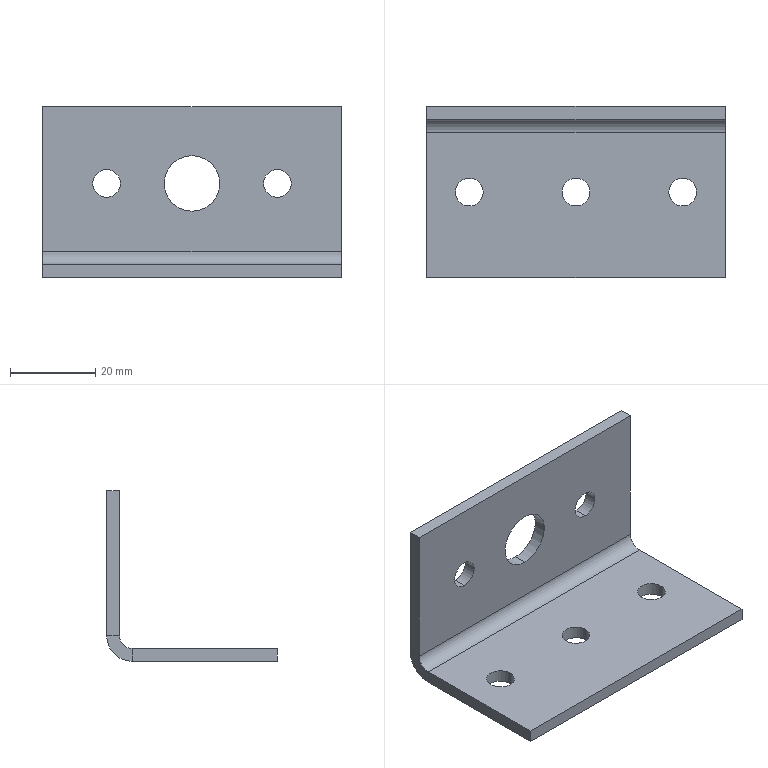Component | SolidWorks | SidePanelAssembly-1_LiftingRingReinforcementPlate-1 | 1 solid | 26 faces | box 70 x 40 x 40 mm | volume 14868 mm3 | cylinder 14 | plane 12 | commonest cylinder face diameters 6.5 x10 13 x2 12 x1 6 x1
STEP:
#1=CARTESIAN_POINT('',(27.472,71.421,-22.766));
#2=VERTEX_POINT('',#1);
#3=CARTESIAN_POINT('',(27.472,71.421,-22.51));
#4=VERTEX_POINT('',#3);
#5=CARTESIAN_POINT('',(27.472,71.421,-22.638));
#6=DIRECTION('',(0.,1.,0.));
#7=DIRECTION('',(0.,0.,1.));
#8=AXIS2_PLACEMENT_3D('',#5,#6,#7);
#9=CIRCLE('',#8,0.128);
#10=EDGE_CURVE('',#2,#4,#9,.T.);
#11=ORIENTED_EDGE('',*,*,#10,.T.);
#12=CARTESIAN_POINT('',(27.472,71.303,-22.51));
#13=VERTEX_POINT('',#12);
#14=CARTESIAN_POINT('',(27.472,71.697,-22.51));
#15=DIRECTION('',(0.,-1.,0.));
#16=VECTOR('',#15,39.37);
#17=LINE('',#14,#16);
#18=EDGE_CURVE('',#4,#13,#17,.T.);
#19=ORIENTED_EDGE('',*,*,#18,.T.);
#20=CARTESIAN_POINT('',(27.472,71.303,-22.766));
#21=VERTEX_POINT('',#20);
#22=CARTESIAN_POINT('',(27.472,71.303,-22.638));
#23=DIRECTION('',(0.,-1.,0.));
#24=DIRECTION('',(0.,0.,-1.));
#25=AXIS2_PLACEMENT_3D('',#22,#23,#24);
#26=CIRCLE('',#25,0.128);
#27=EDGE_CURVE('',#13,#21,#26,.T.);
#28=ORIENTED_EDGE('',*,*,#27,.T.);
#29=CARTESIAN_POINT('',(27.472,71.697,-22.766));
#30=DIRECTION('',(0.,-1.,0.));
#31=VECTOR('',#30,39.37);
#32=LINE('',#29,#31);
#33=EDGE_CURVE('',#2,#21,#32,.T.);
#34=ORIENTED_EDGE('',*,*,#33,.F.);
#35=EDGE_LOOP('',(#11,#19,#28,#34));
#36=FACE_OUTER_BOUND('',#35,.T.);
#37=CARTESIAN_POINT('',(27.472,71.697,-22.638));
#38=DIRECTION('',(0.,-1.,0.));
#39=DIRECTION('',(0.,0.,-1.));
#40=AXIS2_PLACEMENT_3D('',#37,#38,#39);
#41=CYLINDRICAL_SURFACE('',#40,0.128);
#42=ADVANCED_FACE('',(#36),#41,.F.);
#43=CARTESIAN_POINT('',(25.897,71.421,-22.766));
#44=VERTEX_POINT('',#43);
#45=CARTESIAN_POINT('',(25.897,71.421,-22.51));
#46=VERTEX_POINT('',#45);
#47=CARTESIAN_POINT('',(25.897,71.421,-22.638));
#48=DIRECTION('',(0.,1.,0.));
#49=DIRECTION('',(0.,0.,1.));
#50=AXIS2_PLACEMENT_3D('',#47,#48,#49);
#51=CIRCLE('',#50,0.128);
#52=EDGE_CURVE('',#44,#46,#51,.T.);
#53=ORIENTED_EDGE('',*,*,#52,.T.);
#54=CARTESIAN_POINT('',(25.897,71.303,-22.51));
#55=VERTEX_POINT('',#54);
#56=CARTESIAN_POINT('',(25.897,71.697,-22.51));
#57=DIRECTION('',(0.,-1.,0.));
#58=VECTOR('',#57,39.37);
#59=LINE('',#56,#58);
#60=EDGE_CURVE('',#46,#55,#59,.T.);
#61=ORIENTED_EDGE('',*,*,#60,.T.);
#62=CARTESIAN_POINT('',(25.897,71.303,-22.766));
#63=VERTEX_POINT('',#62);
#64=CARTESIAN_POINT('',(25.897,71.303,-22.638));
#65=DIRECTION('',(0.,-1.,0.));
#66=DIRECTION('',(0.,0.,-1.));
#67=AXIS2_PLACEMENT_3D('',#64,#65,#66);
#68=CIRCLE('',#67,0.128);
#69=EDGE_CURVE('',#55,#63,#68,.T.);
#70=ORIENTED_EDGE('',*,*,#69,.T.);
#71=CARTESIAN_POINT('',(25.897,71.697,-22.766));
#72=DIRECTION('',(0.,-1.,0.));
#73=VECTOR('',#72,39.37);
#74=LINE('',#71,#73);
#75=EDGE_CURVE('',#44,#63,#74,.T.);
#76=ORIENTED_EDGE('',*,*,#75,.F.);
#77=EDGE_LOOP('',(#53,#61,#70,#76));
#78=FACE_OUTER_BOUND('',#77,.T.);
#79=CARTESIAN_POINT('',(25.897,71.697,-22.638));
#80=DIRECTION('',(0.,-1.,0.));
#81=DIRECTION('',(0.,0.,-1.));
#82=AXIS2_PLACEMENT_3D('',#79,#80,#81);
#83=CYLINDRICAL_SURFACE('',#82,0.128);
#84=ADVANCED_FACE('',(#78),#83,.F.);
#85=CARTESIAN_POINT('',(27.541,70.634,-23.504));
#86=VERTEX_POINT('',#85);
#87=CARTESIAN_POINT('',(27.797,70.634,-23.504));
#88=VERTEX_POINT('',#87);
#89=CARTESIAN_POINT('',(27.669,70.634,-23.504));
#90=DIRECTION('',(0.,-0.,1.));
#91=DIRECTION('',(0.,-1.,0.));
#92=AXIS2_PLACEMENT_3D('',#89,#90,#91);
#93=CIRCLE('',#92,0.128);
#94=EDGE_CURVE('',#86,#88,#93,.T.);
#95=ORIENTED_EDGE('',*,*,#94,.F.);
#96=CARTESIAN_POINT('',(27.541,70.634,-23.386));
#97=VERTEX_POINT('',#96);
#98=CARTESIAN_POINT('',(27.541,70.634,-23.78));
#99=DIRECTION('',(0.,0.,1.));
#100=VECTOR('',#99,39.37);
#101=LINE('',#98,#100);
#102=EDGE_CURVE('',#86,#97,#101,.T.);
#103=ORIENTED_EDGE('',*,*,#102,.T.);
#104=CARTESIAN_POINT('',(27.797,70.634,-23.386));
#105=VERTEX_POINT('',#104);
#106=CARTESIAN_POINT('',(27.669,70.634,-23.386));
#107=DIRECTION('',(0.,0.,1.));
#108=DIRECTION('',(1.,0.,0.));
#109=AXIS2_PLACEMENT_3D('',#106,#107,#108);
#110=CIRCLE('',#109,0.128);
#111=EDGE_CURVE('',#97,#105,#110,.T.);
#112=ORIENTED_EDGE('',*,*,#111,.T.);
#113=CARTESIAN_POINT('',(27.797,70.634,-23.78));
#114=DIRECTION('',(0.,0.,1.));
#115=VECTOR('',#114,39.37);
#116=LINE('',#113,#115);
#117=EDGE_CURVE('',#88,#105,#116,.T.);
#118=ORIENTED_EDGE('',*,*,#117,.F.);
#119=EDGE_LOOP('',(#95,#103,#112,#118));
#120=FACE_OUTER_BOUND('',#119,.T.);
#121=CARTESIAN_POINT('',(27.669,70.634,-23.78));
#122=DIRECTION('',(0.,0.,1.));
#123=DIRECTION('',(1.,0.,0.));
#124=AXIS2_PLACEMENT_3D('',#121,#122,#123);
#125=CYLINDRICAL_SURFACE('',#124,0.128);
#126=ADVANCED_FACE('',(#120),#125,.F.);
#127=CARTESIAN_POINT('',(26.556,70.634,-23.504));
#128=VERTEX_POINT('',#127);
#129=CARTESIAN_POINT('',(26.812,70.634,-23.504));
#130=VERTEX_POINT('',#129);
#131=CARTESIAN_POINT('',(26.684,70.634,-23.504));
#132=DIRECTION('',(0.,-0.,1.));
#133=DIRECTION('',(0.,-1.,0.));
#134=AXIS2_PLACEMENT_3D('',#131,#132,#133);
#135=CIRCLE('',#134,0.128);
#136=EDGE_CURVE('',#128,#130,#135,.T.);
#137=ORIENTED_EDGE('',*,*,#136,.F.);
#138=CARTESIAN_POINT('',(26.556,70.634,-23.386));
#139=VERTEX_POINT('',#138);
#140=CARTESIAN_POINT('',(26.556,70.634,-23.78));
#141=DIRECTION('',(0.,0.,1.));
#142=VECTOR('',#141,39.37);
#143=LINE('',#140,#142);
#144=EDGE_CURVE('',#128,#139,#143,.T.);
#145=ORIENTED_EDGE('',*,*,#144,.T.);
#146=CARTESIAN_POINT('',(26.812,70.634,-23.386));
#147=VERTEX_POINT('',#146);
#148=CARTESIAN_POINT('',(26.684,70.634,-23.386));
#149=DIRECTION('',(0.,0.,1.));
#150=DIRECTION('',(1.,0.,0.));
#151=AXIS2_PLACEMENT_3D('',#148,#149,#150);
#152=CIRCLE('',#151,0.128);
#153=EDGE_CURVE('',#139,#147,#152,.T.);
#154=ORIENTED_EDGE('',*,*,#153,.T.);
#155=CARTESIAN_POINT('',(26.812,70.634,-23.78));
#156=DIRECTION('',(0.,0.,1.));
#157=VECTOR('',#156,39.37);
#158=LINE('',#155,#157);
#159=EDGE_CURVE('',#130,#147,#158,.T.);
#160=ORIENTED_EDGE('',*,*,#159,.F.);
#161=EDGE_LOOP('',(#137,#145,#154,#160));
#162=FACE_OUTER_BOUND('',#161,.T.);
#163=CARTESIAN_POINT('',(26.684,70.634,-23.78));
#164=DIRECTION('',(0.,0.,1.));
#165=DIRECTION('',(1.,0.,0.));
#166=AXIS2_PLACEMENT_3D('',#163,#164,#165);
#167=CYLINDRICAL_SURFACE('',#166,0.128);
#168=ADVANCED_FACE('',(#162),#167,.F.);
#169=CARTESIAN_POINT('',(25.572,70.634,-23.504));
#170=VERTEX_POINT('',#169);
#171=CARTESIAN_POINT('',(25.828,70.634,-23.504));
#172=VERTEX_POINT('',#171);
#173=CARTESIAN_POINT('',(25.7,70.634,-23.504));
#174=DIRECTION('',(0.,-0.,1.));
#175=DIRECTION('',(0.,-1.,0.));
#176=AXIS2_PLACEMENT_3D('',#173,#174,#175);
#177=CIRCLE('',#176,0.128);
#178=EDGE_CURVE('',#170,#172,#177,.T.);
#179=ORIENTED_EDGE('',*,*,#178,.F.);
#180=CARTESIAN_POINT('',(25.572,70.634,-23.386));
#181=VERTEX_POINT('',#180);
#182=CARTESIAN_POINT('',(25.572,70.634,-23.78));
#183=DIRECTION('',(0.,0.,1.));
#184=VECTOR('',#183,39.37);
#185=LINE('',#182,#184);
#186=EDGE_CURVE('',#170,#181,#185,.T.);
#187=ORIENTED_EDGE('',*,*,#186,.T.);
#188=CARTESIAN_POINT('',(25.828,70.634,-23.386));
#189=VERTEX_POINT('',#188);
#190=CARTESIAN_POINT('',(25.7,70.634,-23.386));
#191=DIRECTION('',(0.,0.,1.));
#192=DIRECTION('',(1.,0.,0.));
#193=AXIS2_PLACEMENT_3D('',#190,#191,#192);
#194=CIRCLE('',#193,0.128);
#195=EDGE_CURVE('',#181,#189,#194,.T.);
#196=ORIENTED_EDGE('',*,*,#195,.T.);
#197=CARTESIAN_POINT('',(25.828,70.634,-23.78));
#198=DIRECTION('',(0.,0.,1.));
#199=VECTOR('',#198,39.37);
#200=LINE('',#197,#199);
#201=EDGE_CURVE('',#172,#189,#200,.T.);
#202=ORIENTED_EDGE('',*,*,#201,.F.);
#203=EDGE_LOOP('',(#179,#187,#196,#202));
#204=FACE_OUTER_BOUND('',#203,.T.);
#205=CARTESIAN_POINT('',(25.7,70.634,-23.78));
#206=DIRECTION('',(0.,0.,1.));
#207=DIRECTION('',(1.,0.,0.));
#208=AXIS2_PLACEMENT_3D('',#205,#206,#207);
#209=CYLINDRICAL_SURFACE('',#208,0.128);
#210=ADVANCED_FACE('',(#204),#209,.F.);
#211=CARTESIAN_POINT('',(26.684,71.303,-22.894));
#212=VERTEX_POINT('',#211);
#213=CARTESIAN_POINT('',(26.684,71.303,-22.382));
#214=VERTEX_POINT('',#213);
#215=CARTESIAN_POINT('',(26.684,71.303,-22.638));
#216=DIRECTION('',(0.,1.,0.));
#217=DIRECTION('',(0.,0.,1.));
#218=AXIS2_PLACEMENT_3D('',#215,#216,#217);
#219=CIRCLE('',#218,0.2559);
#220=EDGE_CURVE('',#212,#214,#219,.T.);
#221=ORIENTED_EDGE('',*,*,#220,.F.);
#222=CARTESIAN_POINT('',(26.684,71.421,-22.894));
#223=VERTEX_POINT('',#222);
#224=CARTESIAN_POINT('',(26.684,71.028,-22.894));
#225=DIRECTION('',(0.,1.,0.));
#226=VECTOR('',#225,39.37);
#227=LINE('',#224,#226);
#228=EDGE_CURVE('',#212,#223,#227,.T.);
#229=ORIENTED_EDGE('',*,*,#228,.T.);
#230=CARTESIAN_POINT('',(26.684,71.421,-22.382));
#231=VERTEX_POINT('',#230);
#232=CARTESIAN_POINT('',(26.684,71.421,-22.638));
#233=DIRECTION('',(0.,1.,0.));
#234=DIRECTION('',(0.,0.,1.));
#235=AXIS2_PLACEMENT_3D('',#232,#233,#234);
#236=CIRCLE('',#235,0.2559);
#237=EDGE_CURVE('',#223,#231,#236,.T.);
#238=ORIENTED_EDGE('',*,*,#237,.T.);
#239=CARTESIAN_POINT('',(26.684,71.028,-22.382));
#240=DIRECTION('',(0.,1.,0.));
#241=VECTOR('',#240,39.37);
#242=LINE('',#239,#241);
#243=EDGE_CURVE('',#214,#231,#242,.T.);
#244=ORIENTED_EDGE('',*,*,#243,.F.);
#245=EDGE_LOOP('',(#221,#229,#238,#244));
#246=FACE_OUTER_BOUND('',#245,.T.);
#247=CARTESIAN_POINT('',(26.684,71.028,-22.638));
#248=DIRECTION('',(0.,1.,0.));
#249=DIRECTION('',(0.,0.,1.));
#250=AXIS2_PLACEMENT_3D('',#247,#248,#249);
#251=CYLINDRICAL_SURFACE('',#250,0.2559);
#252=ADVANCED_FACE('',(#246),#251,.F.);
#253=CARTESIAN_POINT('',(27.472,71.303,-22.638));
#254=DIRECTION('',(0.,-1.,0.));
#255=DIRECTION('',(0.,0.,-1.));
#256=AXIS2_PLACEMENT_3D('',#253,#254,#255);
#257=CIRCLE('',#256,0.128);
#258=EDGE_CURVE('',#21,#13,#257,.T.);
#259=ORIENTED_EDGE('',*,*,#258,.F.);
#260=ORIENTED_EDGE('',*,*,#27,.F.);
#261=EDGE_LOOP('',(#259,#260));
#262=FACE_BOUND('',#261,.T.);
#263=CARTESIAN_POINT('',(25.897,71.303,-22.638));
#264=DIRECTION('',(0.,-1.,0.));
#265=DIRECTION('',(0.,0.,-1.));
#266=AXIS2_PLACEMENT_3D('',#263,#264,#265);
#267=CIRCLE('',#266,0.128);
#268=EDGE_CURVE('',#63,#55,#267,.T.);
#269=ORIENTED_EDGE('',*,*,#268,.F.);
#270=ORIENTED_EDGE('',*,*,#69,.F.);
#271=EDGE_LOOP('',(#269,#270));
#272=FACE_BOUND('',#271,.T.);
#273=CARTESIAN_POINT('',(26.684,71.303,-22.638));
#274=DIRECTION('',(0.,1.,0.));
#275=DIRECTION('',(0.,0.,1.));
#276=AXIS2_PLACEMENT_3D('',#273,#274,#275);
#277=CIRCLE('',#276,0.2559);
#278=EDGE_CURVE('',#214,#212,#277,.T.);
#279=ORIENTED_EDGE('',*,*,#278,.T.);
#280=ORIENTED_EDGE('',*,*,#220,.T.);
#281=EDGE_LOOP('',(#279,#280));
#282=FACE_BOUND('',#281,.T.);
#283=CARTESIAN_POINT('',(28.062,71.303,-23.268));
#284=VERTEX_POINT('',#283);
#285=CARTESIAN_POINT('',(25.306,71.303,-23.268));
#286=VERTEX_POINT('',#285);
#287=CARTESIAN_POINT('',(28.062,71.303,-23.268));
#288=DIRECTION('',(-1.,0.,0.));
#289=VECTOR('',#288,39.37);
#290=LINE('',#287,#289);
#291=EDGE_CURVE('',#284,#286,#290,.T.);
#292=ORIENTED_EDGE('',*,*,#291,.F.);
#293=CARTESIAN_POINT('',(28.062,71.303,-21.929));
#294=VERTEX_POINT('',#293);
#295=CARTESIAN_POINT('',(28.062,71.303,-21.929));
#296=DIRECTION('',(0.,0.,-1.));
#297=VECTOR('',#296,39.37);
#298=LINE('',#295,#297);
#299=EDGE_CURVE('',#294,#284,#298,.T.);
#300=ORIENTED_EDGE('',*,*,#299,.F.);
#301=CARTESIAN_POINT('',(25.306,71.303,-21.929));
#302=VERTEX_POINT('',#301);
#303=CARTESIAN_POINT('',(25.306,71.303,-21.929));
#304=DIRECTION('',(1.,0.,0.));
#305=VECTOR('',#304,39.37);
#306=LINE('',#303,#305);
#307=EDGE_CURVE('',#302,#294,#306,.T.);
#308=ORIENTED_EDGE('',*,*,#307,.F.);
#309=CARTESIAN_POINT('',(25.306,71.303,-21.929));
#310=DIRECTION('',(0.,0.,-1.));
#311=VECTOR('',#310,39.37);
#312=LINE('',#309,#311);
#313=EDGE_CURVE('',#302,#286,#312,.T.);
#314=ORIENTED_EDGE('',*,*,#313,.T.);
#315=EDGE_LOOP('',(#292,#300,#308,#314));
#316=FACE_OUTER_BOUND('',#315,.T.);
#317=CARTESIAN_POINT('',(25.306,71.303,-21.929));
#318=DIRECTION('',(0.,1.,0.));
#319=DIRECTION('',(0.,0.,1.));
#320=AXIS2_PLACEMENT_3D('',#317,#318,#319);
#321=PLANE('',#320);
#322=ADVANCED_FACE('',(#262,#272,#282,#316),#321,.F.);
#323=ORIENTED_EDGE('',*,*,#299,.T.);
#324=CARTESIAN_POINT('',(28.062,71.421,-23.268));
#325=VERTEX_POINT('',#324);
#326=CARTESIAN_POINT('',(28.062,71.303,-23.268));
#327=DIRECTION('',(0.,1.,0.));
#328=VECTOR('',#327,39.37);
#329=LINE('',#326,#328);
#330=EDGE_CURVE('',#284,#325,#329,.T.);
#331=ORIENTED_EDGE('',*,*,#330,.T.);
#332=CARTESIAN_POINT('',(28.062,71.421,-21.929));
#333=VERTEX_POINT('',#332);
#334=CARTESIAN_POINT('',(28.062,71.421,-21.929));
#335=DIRECTION('',(0.,0.,-1.));
#336=VECTOR('',#335,39.37);
#337=LINE('',#334,#336);
#338=EDGE_CURVE('',#333,#325,#337,.T.);
#339=ORIENTED_EDGE('',*,*,#338,.F.);
#340=CARTESIAN_POINT('',(28.062,71.421,-21.929));
#341=DIRECTION('',(0.,-1.,0.));
#342=VECTOR('',#341,39.37);
#343=LINE('',#340,#342);
#344=EDGE_CURVE('',#333,#294,#343,.T.);
#345=ORIENTED_EDGE('',*,*,#344,.T.);
#346=EDGE_LOOP('',(#323,#331,#339,#345));
#347=FACE_OUTER_BOUND('',#346,.T.);
#348=CARTESIAN_POINT('',(28.062,71.421,-21.929));
#349=DIRECTION('',(1.,0.,0.));
#350=DIRECTION('',(0.,0.,-1.));
#351=AXIS2_PLACEMENT_3D('',#348,#349,#350);
#352=PLANE('',#351);
#353=ADVANCED_FACE('',(#347),#352,.T.);
#354=ORIENTED_EDGE('',*,*,#10,.F.);
#355=CARTESIAN_POINT('',(27.472,71.421,-22.638));
#356=DIRECTION('',(0.,1.,0.));
#357=DIRECTION('',(0.,0.,1.));
#358=AXIS2_PLACEMENT_3D('',#355,#356,#357);
#359=CIRCLE('',#358,0.128);
#360=EDGE_CURVE('',#4,#2,#359,.T.);
#361=ORIENTED_EDGE('',*,*,#360,.F.);
#362=EDGE_LOOP('',(#354,#361));
#363=FACE_BOUND('',#362,.T.);
#364=ORIENTED_EDGE('',*,*,#52,.F.);
#365=CARTESIAN_POINT('',(25.897,71.421,-22.638));
#366=DIRECTION('',(0.,1.,0.));
#367=DIRECTION('',(0.,0.,1.));
#368=AXIS2_PLACEMENT_3D('',#365,#366,#367);
#369=CIRCLE('',#368,0.128);
#370=EDGE_CURVE('',#46,#44,#369,.T.);
#371=ORIENTED_EDGE('',*,*,#370,.F.);
#372=EDGE_LOOP('',(#364,#371));
#373=FACE_BOUND('',#372,.T.);
#374=CARTESIAN_POINT('',(26.684,71.421,-22.638));
#375=DIRECTION('',(0.,1.,0.));
#376=DIRECTION('',(0.,0.,1.));
#377=AXIS2_PLACEMENT_3D('',#374,#375,#376);
#378=CIRCLE('',#377,0.2559);
#379=EDGE_CURVE('',#231,#223,#378,.T.);
#380=ORIENTED_EDGE('',*,*,#379,.F.);
#381=ORIENTED_EDGE('',*,*,#237,.F.);
#382=EDGE_LOOP('',(#380,#381));
#383=FACE_BOUND('',#382,.T.);
#384=ORIENTED_EDGE('',*,*,#338,.T.);
#385=CARTESIAN_POINT('',(25.306,71.421,-23.268));
#386=VERTEX_POINT('',#385);
#387=CARTESIAN_POINT('',(28.062,71.421,-23.268));
#388=DIRECTION('',(-1.,0.,0.));
#389=VECTOR('',#388,39.37);
#390=LINE('',#387,#389);
#391=EDGE_CURVE('',#325,#386,#390,.T.);
#392=ORIENTED_EDGE('',*,*,#391,.T.);
#393=CARTESIAN_POINT('',(25.306,71.421,-21.929));
#394=VERTEX_POINT('',#393);
#395=CARTESIAN_POINT('',(25.306,71.421,-21.929));
#396=DIRECTION('',(0.,0.,-1.));
#397=VECTOR('',#396,39.37);
#398=LINE('',#395,#397);
#399=EDGE_CURVE('',#394,#386,#398,.T.);
#400=ORIENTED_EDGE('',*,*,#399,.F.);
#401=CARTESIAN_POINT('',(25.306,71.421,-21.929));
#402=DIRECTION('',(1.,0.,0.));
#403=VECTOR('',#402,39.37);
#404=LINE('',#401,#403);
#405=EDGE_CURVE('',#394,#333,#404,.T.);
#406=ORIENTED_EDGE('',*,*,#405,.T.);
#407=EDGE_LOOP('',(#384,#392,#400,#406));
#408=FACE_OUTER_BOUND('',#407,.T.);
#409=CARTESIAN_POINT('',(25.306,71.421,-21.929));
#410=DIRECTION('',(0.,1.,0.));
#411=DIRECTION('',(0.,0.,1.));
#412=AXIS2_PLACEMENT_3D('',#409,#410,#411);
#413=PLANE('',#412);
#414=ADVANCED_FACE('',(#363,#373,#383,#408),#413,.T.);
#415=CARTESIAN_POINT('',(25.306,71.303,-23.268));
#416=DIRECTION('',(0.,1.,0.));
#417=VECTOR('',#416,39.37);
#418=LINE('',#415,#417);
#419=EDGE_CURVE('',#286,#386,#418,.T.);
#420=ORIENTED_EDGE('',*,*,#419,.F.);
#421=ORIENTED_EDGE('',*,*,#313,.F.);
#422=CARTESIAN_POINT('',(25.306,71.303,-21.929));
#423=DIRECTION('',(0.,1.,0.));
#424=VECTOR('',#423,39.37);
#425=LINE('',#422,#424);
#426=EDGE_CURVE('',#302,#394,#425,.T.);
#427=ORIENTED_EDGE('',*,*,#426,.T.);
#428=ORIENTED_EDGE('',*,*,#399,.T.);
#429=EDGE_LOOP('',(#420,#421,#427,#428));
#430=FACE_OUTER_BOUND('',#429,.T.);
#431=CARTESIAN_POINT('',(25.306,71.303,-21.929));
#432=DIRECTION('',(-1.,0.,0.));
#433=DIRECTION('',(0.,0.,1.));
#434=AXIS2_PLACEMENT_3D('',#431,#432,#433);
#435=PLANE('',#434);
#436=ADVANCED_FACE('',(#430),#435,.T.);
#437=ORIENTED_EDGE('',*,*,#307,.T.);
#438=ORIENTED_EDGE('',*,*,#344,.F.);
#439=ORIENTED_EDGE('',*,*,#405,.F.);
#440=ORIENTED_EDGE('',*,*,#426,.F.);
#441=EDGE_LOOP('',(#437,#438,#439,#440));
#442=FACE_OUTER_BOUND('',#441,.T.);
#443=CARTESIAN_POINT('',(28.062,71.303,-21.929));
#444=DIRECTION('',(0.,0.,-1.));
#445=DIRECTION('',(-1.,0.,0.));
#446=AXIS2_PLACEMENT_3D('',#443,#444,#445);
#447=PLANE('',#446);
#448=ADVANCED_FACE('',(#442),#447,.F.);
#449=CARTESIAN_POINT('',(25.306,71.185,-23.386));
#450=VERTEX_POINT('',#449);
#451=CARTESIAN_POINT('',(25.306,71.185,-23.504));
#452=VERTEX_POINT('',#451);
#453=CARTESIAN_POINT('',(25.306,71.185,-23.504));
#454=DIRECTION('',(0.,0.,-1.));
#455=VECTOR('',#454,39.37);
#456=LINE('',#453,#455);
#457=EDGE_CURVE('',#450,#452,#456,.T.);
#458=ORIENTED_EDGE('',*,*,#457,.F.);
#459=CARTESIAN_POINT('',(25.306,71.185,-23.268));
#460=DIRECTION('',(-1.,0.,0.));
#461=DIRECTION('',(0.,0.,-1.));
#462=AXIS2_PLACEMENT_3D('',#459,#460,#461);
#463=CIRCLE('',#462,0.1181);
#464=EDGE_CURVE('',#286,#450,#463,.T.);
#465=ORIENTED_EDGE('',*,*,#464,.F.);
#466=ORIENTED_EDGE('',*,*,#419,.T.);
#467=CARTESIAN_POINT('',(25.306,71.185,-23.268));
#468=DIRECTION('',(-1.,0.,0.));
#469=DIRECTION('',(0.,0.,-1.));
#470=AXIS2_PLACEMENT_3D('',#467,#468,#469);
#471=CIRCLE('',#470,0.2362);
#472=EDGE_CURVE('',#386,#452,#471,.T.);
#473=ORIENTED_EDGE('',*,*,#472,.T.);
#474=EDGE_LOOP('',(#458,#465,#466,#473));
#475=FACE_OUTER_BOUND('',#474,.T.);
#476=CARTESIAN_POINT('',(25.306,71.185,-23.268));
#477=DIRECTION('',(-1.,0.,0.));
#478=DIRECTION('',(0.,0.,1.));
#479=AXIS2_PLACEMENT_3D('',#476,#477,#478);
#480=PLANE('',#479);
#481=ADVANCED_FACE('',(#475),#480,.T.);
#482=ORIENTED_EDGE('',*,*,#391,.F.);
#483=CARTESIAN_POINT('',(28.062,71.185,-23.504));
#484=VERTEX_POINT('',#483);
#485=CARTESIAN_POINT('',(28.062,71.185,-23.268));
#486=DIRECTION('',(1.,0.,0.));
#487=DIRECTION('',(0.,0.,-1.));
#488=AXIS2_PLACEMENT_3D('',#485,#486,#487);
#489=CIRCLE('',#488,0.2362);
#490=EDGE_CURVE('',#484,#325,#489,.T.);
#491=ORIENTED_EDGE('',*,*,#490,.F.);
#492=CARTESIAN_POINT('',(25.306,71.185,-23.504));
#493=DIRECTION('',(-1.,0.,0.));
#494=VECTOR('',#493,39.37);
#495=LINE('',#492,#494);
#496=EDGE_CURVE('',#484,#452,#495,.T.);
#497=ORIENTED_EDGE('',*,*,#496,.T.);
#498=ORIENTED_EDGE('',*,*,#472,.F.);
#499=EDGE_LOOP('',(#482,#491,#497,#498));
#500=FACE_OUTER_BOUND('',#499,.T.);
#501=CARTESIAN_POINT('',(28.062,71.185,-23.268));
#502=DIRECTION('',(1.,0.,0.));
#503=DIRECTION('',(0.,0.,-1.));
#504=AXIS2_PLACEMENT_3D('',#501,#502,#503);
#505=CYLINDRICAL_SURFACE('',#504,0.2362);
#506=ADVANCED_FACE('',(#500),#505,.T.);
#507=CARTESIAN_POINT('',(28.062,71.185,-23.386));
#508=VERTEX_POINT('',#507);
#509=CARTESIAN_POINT('',(28.062,71.185,-23.268));
#510=DIRECTION('',(1.,0.,0.));
#511=DIRECTION('',(0.,0.,-1.));
#512=AXIS2_PLACEMENT_3D('',#509,#510,#511);
#513=CIRCLE('',#512,0.1181);
#514=EDGE_CURVE('',#508,#284,#513,.T.);
#515=ORIENTED_EDGE('',*,*,#514,.F.);
#516=CARTESIAN_POINT('',(28.062,71.185,-23.386));
#517=DIRECTION('',(0.,0.,-1.));
#518=VECTOR('',#517,39.37);
#519=LINE('',#516,#518);
#520=EDGE_CURVE('',#508,#484,#519,.T.);
#521=ORIENTED_EDGE('',*,*,#520,.T.);
#522=ORIENTED_EDGE('',*,*,#490,.T.);
#523=ORIENTED_EDGE('',*,*,#330,.F.);
#524=EDGE_LOOP('',(#515,#521,#522,#523));
#525=FACE_OUTER_BOUND('',#524,.T.);
#526=CARTESIAN_POINT('',(28.062,71.185,-23.268));
#527=DIRECTION('',(-1.,0.,0.));
#528=DIRECTION('',(0.,0.,1.));
#529=AXIS2_PLACEMENT_3D('',#526,#527,#528);
#530=PLANE('',#529);
#531=ADVANCED_FACE('',(#525),#530,.F.);
#532=ORIENTED_EDGE('',*,*,#291,.T.);
#533=ORIENTED_EDGE('',*,*,#464,.T.);
#534=CARTESIAN_POINT('',(25.306,71.185,-23.386));
#535=DIRECTION('',(1.,0.,0.));
#536=VECTOR('',#535,39.37);
#537=LINE('',#534,#536);
#538=EDGE_CURVE('',#450,#508,#537,.T.);
#539=ORIENTED_EDGE('',*,*,#538,.T.);
#540=ORIENTED_EDGE('',*,*,#514,.T.);
#541=EDGE_LOOP('',(#532,#533,#539,#540));
#542=FACE_OUTER_BOUND('',#541,.T.);
#543=CARTESIAN_POINT('',(28.062,71.185,-23.268));
#544=DIRECTION('',(1.,0.,0.));
#545=DIRECTION('',(0.,0.,-1.));
#546=AXIS2_PLACEMENT_3D('',#543,#544,#545);
#547=CYLINDRICAL_SURFACE('',#546,0.1181);
#548=ADVANCED_FACE('',(#542),#547,.F.);
#549=ORIENTED_EDGE('',*,*,#457,.T.);
#550=CARTESIAN_POINT('',(25.306,69.846,-23.504));
#551=VERTEX_POINT('',#550);
#552=CARTESIAN_POINT('',(25.306,69.846,-23.504));
#553=DIRECTION('',(0.,1.,0.));
#554=VECTOR('',#553,39.37);
#555=LINE('',#552,#554);
#556=EDGE_CURVE('',#551,#452,#555,.T.);
#557=ORIENTED_EDGE('',*,*,#556,.F.);
#558=CARTESIAN_POINT('',(25.306,69.846,-23.386));
#559=VERTEX_POINT('',#558);
#560=CARTESIAN_POINT('',(25.306,69.846,-23.504));
#561=DIRECTION('',(0.,-0.,1.));
#562=VECTOR('',#561,39.37);
#563=LINE('',#560,#562);
#564=EDGE_CURVE('',#551,#559,#563,.T.);
#565=ORIENTED_EDGE('',*,*,#564,.T.);
#566=CARTESIAN_POINT('',(25.306,71.303,-23.386));
#567=DIRECTION('',(0.,1.,0.));
#568=VECTOR('',#567,39.37);
#569=LINE('',#566,#568);
#570=EDGE_CURVE('',#559,#450,#569,.T.);
#571=ORIENTED_EDGE('',*,*,#570,.T.);
#572=EDGE_LOOP('',(#549,#557,#565,#571));
#573=FACE_OUTER_BOUND('',#572,.T.);
#574=CARTESIAN_POINT('',(25.306,71.303,-23.504));
#575=DIRECTION('',(1.,0.,0.));
#576=DIRECTION('',(0.,0.,-1.));
#577=AXIS2_PLACEMENT_3D('',#574,#575,#576);
#578=PLANE('',#577);
#579=ADVANCED_FACE('',(#573),#578,.F.);
#580=ORIENTED_EDGE('',*,*,#520,.F.);
#581=CARTESIAN_POINT('',(28.062,69.846,-23.386));
#582=VERTEX_POINT('',#581);
#583=CARTESIAN_POINT('',(28.062,69.846,-23.386));
#584=DIRECTION('',(0.,-1.,-0.));
#585=VECTOR('',#584,39.37);
#586=LINE('',#583,#585);
#587=EDGE_CURVE('',#508,#582,#586,.T.);
#588=ORIENTED_EDGE('',*,*,#587,.T.);
#589=CARTESIAN_POINT('',(28.062,69.846,-23.504));
#590=VERTEX_POINT('',#589);
#591=CARTESIAN_POINT('',(28.062,69.846,-23.504));
#592=DIRECTION('',(0.,-0.,1.));
#593=VECTOR('',#592,39.37);
#594=LINE('',#591,#593);
#595=EDGE_CURVE('',#590,#582,#594,.T.);
#596=ORIENTED_EDGE('',*,*,#595,.F.);
#597=CARTESIAN_POINT('',(28.062,69.846,-23.504));
#598=DIRECTION('',(0.,-1.,-0.));
#599=VECTOR('',#598,39.37);
#600=LINE('',#597,#599);
#601=EDGE_CURVE('',#484,#590,#600,.T.);
#602=ORIENTED_EDGE('',*,*,#601,.F.);
#603=EDGE_LOOP('',(#580,#588,#596,#602));
#604=FACE_OUTER_BOUND('',#603,.T.);
#605=CARTESIAN_POINT('',(28.062,69.846,-23.504));
#606=DIRECTION('',(-1.,0.,0.));
#607=DIRECTION('',(0.,0.,1.));
#608=AXIS2_PLACEMENT_3D('',#605,#606,#607);
#609=PLANE('',#608);
#610=ADVANCED_FACE('',(#604),#609,.F.);
#611=CARTESIAN_POINT('',(26.684,70.634,-23.504));
#612=DIRECTION('',(0.,-0.,1.));
#613=DIRECTION('',(0.,-1.,0.));
#614=AXIS2_PLACEMENT_3D('',#611,#612,#613);
#615=CIRCLE('',#614,0.128);
#616=EDGE_CURVE('',#130,#128,#615,.T.);
#617=ORIENTED_EDGE('',*,*,#616,.T.);
#618=ORIENTED_EDGE('',*,*,#136,.T.);
#619=EDGE_LOOP('',(#617,#618));
#620=FACE_BOUND('',#619,.T.);
#621=CARTESIAN_POINT('',(25.7,70.634,-23.504));
#622=DIRECTION('',(0.,-0.,1.));
#623=DIRECTION('',(0.,-1.,0.));
#624=AXIS2_PLACEMENT_3D('',#621,#622,#623);
#625=CIRCLE('',#624,0.128);
#626=EDGE_CURVE('',#172,#170,#625,.T.);
#627=ORIENTED_EDGE('',*,*,#626,.T.);
#628=ORIENTED_EDGE('',*,*,#178,.T.);
#629=EDGE_LOOP('',(#627,#628));
#630=FACE_BOUND('',#629,.T.);
#631=ORIENTED_EDGE('',*,*,#496,.F.);
#632=ORIENTED_EDGE('',*,*,#601,.T.);
#633=CARTESIAN_POINT('',(25.306,69.846,-23.504));
#634=DIRECTION('',(-1.,0.,0.));
#635=VECTOR('',#634,39.37);
#636=LINE('',#633,#635);
#637=EDGE_CURVE('',#590,#551,#636,.T.);
#638=ORIENTED_EDGE('',*,*,#637,.T.);
#639=ORIENTED_EDGE('',*,*,#556,.T.);
#640=EDGE_LOOP('',(#631,#632,#638,#639));
#641=FACE_OUTER_BOUND('',#640,.T.);
#642=CARTESIAN_POINT('',(27.669,70.634,-23.504));
#643=DIRECTION('',(0.,-0.,1.));
#644=DIRECTION('',(0.,-1.,0.));
#645=AXIS2_PLACEMENT_3D('',#642,#643,#644);
#646=CIRCLE('',#645,0.128);
#647=EDGE_CURVE('',#88,#86,#646,.T.);
#648=ORIENTED_EDGE('',*,*,#647,.T.);
#649=ORIENTED_EDGE('',*,*,#94,.T.);
#650=EDGE_LOOP('',(#648,#649));
#651=FACE_BOUND('',#650,.T.);
#652=CARTESIAN_POINT('',(25.306,69.846,-23.504));
#653=DIRECTION('',(0.,-0.,1.));
#654=DIRECTION('',(0.,-1.,-0.));
#655=AXIS2_PLACEMENT_3D('',#652,#653,#654);
#656=PLANE('',#655);
#657=ADVANCED_FACE('',(#620,#630,#641,#651),#656,.F.);
#658=CARTESIAN_POINT('',(26.684,70.634,-23.386));
#659=DIRECTION('',(0.,0.,1.));
#660=DIRECTION('',(1.,0.,0.));
#661=AXIS2_PLACEMENT_3D('',#658,#659,#660);
#662=CIRCLE('',#661,0.128);
#663=EDGE_CURVE('',#147,#139,#662,.T.);
#664=ORIENTED_EDGE('',*,*,#663,.F.);
#665=ORIENTED_EDGE('',*,*,#153,.F.);
#666=EDGE_LOOP('',(#664,#665));
#667=FACE_BOUND('',#666,.T.);
#668=CARTESIAN_POINT('',(25.7,70.634,-23.386));
#669=DIRECTION('',(0.,0.,1.));
#670=DIRECTION('',(1.,0.,0.));
#671=AXIS2_PLACEMENT_3D('',#668,#669,#670);
#672=CIRCLE('',#671,0.128);
#673=EDGE_CURVE('',#189,#181,#672,.T.);
#674=ORIENTED_EDGE('',*,*,#673,.F.);
#675=ORIENTED_EDGE('',*,*,#195,.F.);
#676=EDGE_LOOP('',(#674,#675));
#677=FACE_BOUND('',#676,.T.);
#678=ORIENTED_EDGE('',*,*,#587,.F.);
#679=ORIENTED_EDGE('',*,*,#538,.F.);
#680=ORIENTED_EDGE('',*,*,#570,.F.);
#681=CARTESIAN_POINT('',(25.306,69.846,-23.386));
#682=DIRECTION('',(-1.,0.,0.));
#683=VECTOR('',#682,39.37);
#684=LINE('',#681,#683);
#685=EDGE_CURVE('',#582,#559,#684,.T.);
#686=ORIENTED_EDGE('',*,*,#685,.F.);
#687=EDGE_LOOP('',(#678,#679,#680,#686));
#688=FACE_OUTER_BOUND('',#687,.T.);
#689=CARTESIAN_POINT('',(27.669,70.634,-23.386));
#690=DIRECTION('',(0.,0.,1.));
#691=DIRECTION('',(1.,0.,0.));
#692=AXIS2_PLACEMENT_3D('',#689,#690,#691);
#693=CIRCLE('',#692,0.128);
#694=EDGE_CURVE('',#105,#97,#693,.T.);
#695=ORIENTED_EDGE('',*,*,#694,.F.);
#696=ORIENTED_EDGE('',*,*,#111,.F.);
#697=EDGE_LOOP('',(#695,#696));
#698=FACE_BOUND('',#697,.T.);
#699=CARTESIAN_POINT('',(25.306,69.846,-23.386));
#700=DIRECTION('',(0.,-0.,1.));
#701=DIRECTION('',(0.,-1.,-0.));
#702=AXIS2_PLACEMENT_3D('',#699,#700,#701);
#703=PLANE('',#702);
#704=ADVANCED_FACE('',(#667,#677,#688,#698),#703,.T.);
#705=ORIENTED_EDGE('',*,*,#685,.T.);
#706=ORIENTED_EDGE('',*,*,#564,.F.);
#707=ORIENTED_EDGE('',*,*,#637,.F.);
#708=ORIENTED_EDGE('',*,*,#595,.T.);
#709=EDGE_LOOP('',(#705,#706,#707,#708));
#710=FACE_OUTER_BOUND('',#709,.T.);
#711=CARTESIAN_POINT('',(25.306,69.846,-23.504));
#712=DIRECTION('',(0.,1.,0.));
#713=DIRECTION('',(0.,-0.,1.));
#714=AXIS2_PLACEMENT_3D('',#711,#712,#713);
#715=PLANE('',#714);
#716=ADVANCED_FACE('',(#710),#715,.F.);
#717=ORIENTED_EDGE('',*,*,#228,.F.);
#718=ORIENTED_EDGE('',*,*,#278,.F.);
#719=ORIENTED_EDGE('',*,*,#243,.T.);
#720=ORIENTED_EDGE('',*,*,#379,.T.);
#721=EDGE_LOOP('',(#717,#718,#719,#720));
#722=FACE_OUTER_BOUND('',#721,.T.);
#723=CARTESIAN_POINT('',(26.684,71.028,-22.638));
#724=DIRECTION('',(0.,1.,0.));
#725=DIRECTION('',(0.,0.,1.));
#726=AXIS2_PLACEMENT_3D('',#723,#724,#725);
#727=CYLINDRICAL_SURFACE('',#726,0.2559);
#728=ADVANCED_FACE('',(#722),#727,.F.);
#729=ORIENTED_EDGE('',*,*,#186,.F.);
#730=ORIENTED_EDGE('',*,*,#626,.F.);
#731=ORIENTED_EDGE('',*,*,#201,.T.);
#732=ORIENTED_EDGE('',*,*,#673,.T.);
#733=EDGE_LOOP('',(#729,#730,#731,#732));
#734=FACE_OUTER_BOUND('',#733,.T.);
#735=CARTESIAN_POINT('',(25.7,70.634,-23.78));
#736=DIRECTION('',(0.,0.,1.));
#737=DIRECTION('',(1.,0.,0.));
#738=AXIS2_PLACEMENT_3D('',#735,#736,#737);
#739=CYLINDRICAL_SURFACE('',#738,0.128);
#740=ADVANCED_FACE('',(#734),#739,.F.);
#741=ORIENTED_EDGE('',*,*,#144,.F.);
#742=ORIENTED_EDGE('',*,*,#616,.F.);
#743=ORIENTED_EDGE('',*,*,#159,.T.);
#744=ORIENTED_EDGE('',*,*,#663,.T.);
#745=EDGE_LOOP('',(#741,#742,#743,#744));
#746=FACE_OUTER_BOUND('',#745,.T.);
#747=CARTESIAN_POINT('',(26.684,70.634,-23.78));
#748=DIRECTION('',(0.,0.,1.));
#749=DIRECTION('',(1.,0.,0.));
#750=AXIS2_PLACEMENT_3D('',#747,#748,#749);
#751=CYLINDRICAL_SURFACE('',#750,0.128);
#752=ADVANCED_FACE('',(#746),#751,.F.);
#753=ORIENTED_EDGE('',*,*,#102,.F.);
#754=ORIENTED_EDGE('',*,*,#647,.F.);
#755=ORIENTED_EDGE('',*,*,#117,.T.);
#756=ORIENTED_EDGE('',*,*,#694,.T.);
#757=EDGE_LOOP('',(#753,#754,#755,#756));
#758=FACE_OUTER_BOUND('',#757,.T.);
#759=CARTESIAN_POINT('',(27.669,70.634,-23.78));
#760=DIRECTION('',(0.,0.,1.));
#761=DIRECTION('',(1.,0.,0.));
#762=AXIS2_PLACEMENT_3D('',#759,#760,#761);
#763=CYLINDRICAL_SURFACE('',#762,0.128);
#764=ADVANCED_FACE('',(#758),#763,.F.);
#765=ORIENTED_EDGE('',*,*,#60,.F.);
#766=ORIENTED_EDGE('',*,*,#370,.T.);
#767=ORIENTED_EDGE('',*,*,#75,.T.);
#768=ORIENTED_EDGE('',*,*,#268,.T.);
#769=EDGE_LOOP('',(#765,#766,#767,#768));
#770=FACE_OUTER_BOUND('',#769,.T.);
#771=CARTESIAN_POINT('',(25.897,71.697,-22.638));
#772=DIRECTION('',(0.,-1.,0.));
#773=DIRECTION('',(0.,0.,-1.));
#774=AXIS2_PLACEMENT_3D('',#771,#772,#773);
#775=CYLINDRICAL_SURFACE('',#774,0.128);
#776=ADVANCED_FACE('',(#770),#775,.F.);
#777=ORIENTED_EDGE('',*,*,#18,.F.);
#778=ORIENTED_EDGE('',*,*,#360,.T.);
#779=ORIENTED_EDGE('',*,*,#33,.T.);
#780=ORIENTED_EDGE('',*,*,#258,.T.);
#781=EDGE_LOOP('',(#777,#778,#779,#780));
#782=FACE_OUTER_BOUND('',#781,.T.);
#783=CARTESIAN_POINT('',(27.472,71.697,-22.638));
#784=DIRECTION('',(0.,-1.,0.));
#785=DIRECTION('',(0.,0.,-1.));
#786=AXIS2_PLACEMENT_3D('',#783,#784,#785);
#787=CYLINDRICAL_SURFACE('',#786,0.128);
#788=ADVANCED_FACE('',(#782),#787,.F.);
#789=CLOSED_SHELL('',(#42,#84,#126,#168,#210,#252,#322,#353,#414,#436,#448,#481,#506,#531,#548,#579,#610,#657,#704,#716,#728,#740,#752,#764,#776,#788));
#790=MANIFOLD_SOLID_BREP('',#789);
#791=CARTESIAN_POINT('',(0.,0.,0.));
#792=DIRECTION('',(0.,0.,1.));
#793=DIRECTION('',(1.,0.,0.));
#794=AXIS2_PLACEMENT_3D('',#791,#792,#793);
#795=(LENGTH_UNIT()NAMED_UNIT(*)SI_UNIT($,.METRE.));
#796=LENGTH_MEASURE_WITH_UNIT(LENGTH_MEASURE(0.0254),#795);
#797=DIMENSIONAL_EXPONENTS(1.,0.,0.,0.,0.,0.,0.);
#798=(CONVERSION_BASED_UNIT('',#796)LENGTH_UNIT()NAMED_UNIT(#797));
#799=UNCERTAINTY_MEASURE_WITH_UNIT(LENGTH_MEASURE(0.00001),#798,'','');
#800=(NAMED_UNIT(*)PLANE_ANGLE_UNIT()SI_UNIT($,.RADIAN.));
#801=(NAMED_UNIT(*)SI_UNIT($,.STERADIAN.)SOLID_ANGLE_UNIT());
#802=(GEOMETRIC_REPRESENTATION_CONTEXT(3)GLOBAL_UNCERTAINTY_ASSIGNED_CONTEXT((#799))GLOBAL_UNIT_ASSIGNED_CONTEXT((#798,#800,#801))REPRESENTATION_CONTEXT('',''));
#803=ADVANCED_BREP_SHAPE_REPRESENTATION('',(#790,#794),#802);
#804=COLOUR_RGB('',0.7922,0.8196,0.9333);
#805=FILL_AREA_STYLE_COLOUR('',#804);
#806=FILL_AREA_STYLE('',(#805));
#807=SURFACE_STYLE_FILL_AREA(#806);
#808=SURFACE_SIDE_STYLE('',(#807));
#809=SURFACE_STYLE_USAGE(.BOTH.,#808);
#810=PRESENTATION_STYLE_ASSIGNMENT((#809));
#811=STYLED_ITEM('',(#810),#790);
#812=PRESENTATION_LAYER_ASSIGNMENT('','',(#811));
#813=(LENGTH_UNIT()NAMED_UNIT(*)SI_UNIT($,.METRE.));
#814=LENGTH_MEASURE_WITH_UNIT(LENGTH_MEASURE(0.0254),#813);
#815=DIMENSIONAL_EXPONENTS(1.,0.,0.,0.,0.,0.,0.);
#816=(CONVERSION_BASED_UNIT('',#814)LENGTH_UNIT()NAMED_UNIT(#815));
#817=UNCERTAINTY_MEASURE_WITH_UNIT(LENGTH_MEASURE(0.00001),#816,'','');
#818=(NAMED_UNIT(*)PLANE_ANGLE_UNIT()SI_UNIT($,.RADIAN.));
#819=(NAMED_UNIT(*)SI_UNIT($,.STERADIAN.)SOLID_ANGLE_UNIT());
#820=(GEOMETRIC_REPRESENTATION_CONTEXT(3)GLOBAL_UNCERTAINTY_ASSIGNED_CONTEXT((#817))GLOBAL_UNIT_ASSIGNED_CONTEXT((#816,#818,#819))REPRESENTATION_CONTEXT('',''));
#821=MECHANICAL_DESIGN_GEOMETRIC_PRESENTATION_REPRESENTATION('',(#811),#820);